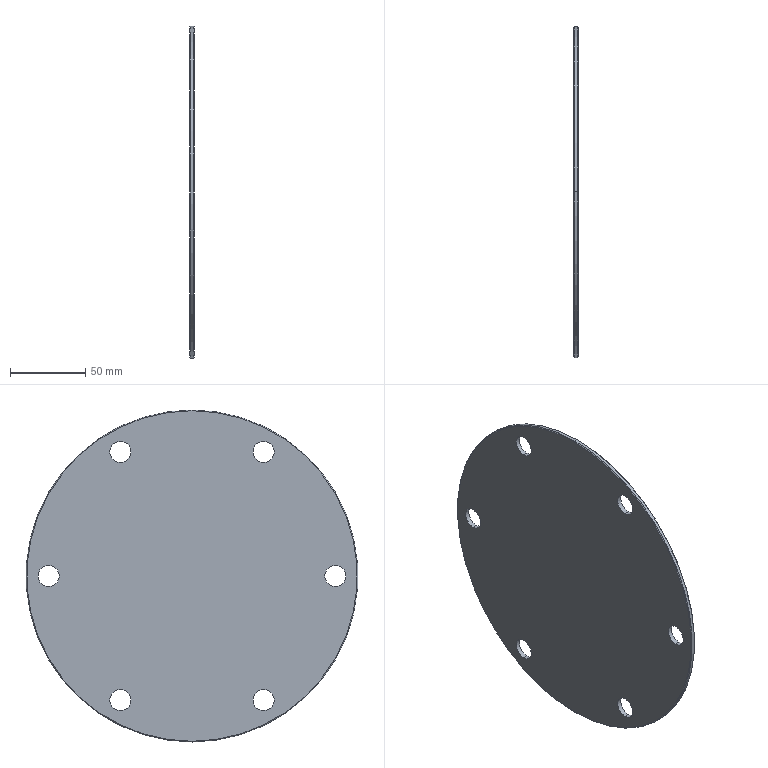Component | SolidWorks | YC1-200-01-11BodySideCover-1 | 1 solid | 20 faces | box 3 x 220 x 220 mm | volume 111096 mm3 | cylinder 14 | cone 4 | plane 2 | commonest cylinder face diameters 14 x12 220 x2 | material Plain Carbon Steel
STEP:
#1=COLOUR_RGB('',0.7922,0.8196,0.9333);
#2=FILL_AREA_STYLE_COLOUR('',#1);
#3=FILL_AREA_STYLE('',(#2));
#4=SURFACE_STYLE_FILL_AREA(#3);
#5=SURFACE_SIDE_STYLE('',(#4));
#6=SURFACE_STYLE_USAGE(.BOTH.,#5);
#7=PRESENTATION_STYLE_ASSIGNMENT((#6));
#8=CARTESIAN_POINT('',(-26.378,131.693,-29.508));
#9=VERTEX_POINT('',#8);
#10=CARTESIAN_POINT('',(-26.378,131.693,-38.13));
#11=VERTEX_POINT('',#10);
#12=CARTESIAN_POINT('',(-26.378,131.693,-33.819));
#13=DIRECTION('',(-1.,0.,0.));
#14=DIRECTION('',(0.,0.,1.));
#15=AXIS2_PLACEMENT_3D('',#12,#13,#14);
#16=CIRCLE('',#15,4.311);
#17=EDGE_CURVE('',#9,#11,#16,.T.);
#18=ORIENTED_EDGE('',*,*,#17,.T.);
#19=CARTESIAN_POINT('',(-26.398,131.693,-38.15));
#20=VERTEX_POINT('',#19);
#21=CARTESIAN_POINT('',(-26.398,131.693,-38.15));
#22=DIRECTION('',(-0.7071,0.,-0.7071));
#23=VECTOR('',#22,39.37);
#24=LINE('',#21,#23);
#25=EDGE_CURVE('',#11,#20,#24,.T.);
#26=ORIENTED_EDGE('',*,*,#25,.T.);
#27=CARTESIAN_POINT('',(-26.398,131.693,-29.488));
#28=VERTEX_POINT('',#27);
#29=CARTESIAN_POINT('',(-26.398,131.693,-33.819));
#30=DIRECTION('',(1.,0.,0.));
#31=DIRECTION('',(0.,0.,1.));
#32=AXIS2_PLACEMENT_3D('',#29,#30,#31);
#33=CIRCLE('',#32,4.331);
#34=EDGE_CURVE('',#20,#28,#33,.T.);
#35=ORIENTED_EDGE('',*,*,#34,.T.);
#36=CARTESIAN_POINT('',(-26.398,131.693,-29.488));
#37=DIRECTION('',(-0.7071,0.,0.7071));
#38=VECTOR('',#37,39.37);
#39=LINE('',#36,#38);
#40=EDGE_CURVE('',#9,#28,#39,.T.);
#41=ORIENTED_EDGE('',*,*,#40,.F.);
#42=EDGE_LOOP('',(#18,#26,#35,#41));
#43=FACE_OUTER_BOUND('',#42,.T.);
#44=CARTESIAN_POINT('',(-26.398,131.693,-33.819));
#45=DIRECTION('',(-1.,0.,0.));
#46=DIRECTION('',(0.,0.,1.));
#47=AXIS2_PLACEMENT_3D('',#44,#45,#46);
#48=CONICAL_SURFACE('',#47,4.331,0.7854);
#49=ADVANCED_FACE('',(#43),#48,.T.);
#50=CARTESIAN_POINT('',(-26.378,133.563,-36.782));
#51=VERTEX_POINT('',#50);
#52=CARTESIAN_POINT('',(-26.378,133.563,-37.334));
#53=VERTEX_POINT('',#52);
#54=CARTESIAN_POINT('',(-26.378,133.563,-37.058));
#55=DIRECTION('',(1.,0.,0.));
#56=DIRECTION('',(0.,0.,1.));
#57=AXIS2_PLACEMENT_3D('',#54,#55,#56);
#58=CIRCLE('',#57,0.2756);
#59=EDGE_CURVE('',#51,#53,#58,.T.);
#60=ORIENTED_EDGE('',*,*,#59,.T.);
#61=CARTESIAN_POINT('',(-26.496,133.563,-37.334));
#62=VERTEX_POINT('',#61);
#63=CARTESIAN_POINT('',(-26.496,133.563,-37.334));
#64=DIRECTION('',(-1.,0.,0.));
#65=VECTOR('',#64,39.37);
#66=LINE('',#63,#65);
#67=EDGE_CURVE('',#53,#62,#66,.T.);
#68=ORIENTED_EDGE('',*,*,#67,.T.);
#69=CARTESIAN_POINT('',(-26.496,133.563,-36.782));
#70=VERTEX_POINT('',#69);
#71=CARTESIAN_POINT('',(-26.496,133.563,-37.058));
#72=DIRECTION('',(1.,0.,0.));
#73=DIRECTION('',(0.,0.,1.));
#74=AXIS2_PLACEMENT_3D('',#71,#72,#73);
#75=CIRCLE('',#74,0.2756);
#76=EDGE_CURVE('',#70,#62,#75,.T.);
#77=ORIENTED_EDGE('',*,*,#76,.F.);
#78=CARTESIAN_POINT('',(-26.496,133.563,-36.782));
#79=DIRECTION('',(-1.,0.,0.));
#80=VECTOR('',#79,39.37);
#81=LINE('',#78,#80);
#82=EDGE_CURVE('',#51,#70,#81,.T.);
#83=ORIENTED_EDGE('',*,*,#82,.F.);
#84=EDGE_LOOP('',(#60,#68,#77,#83));
#85=FACE_OUTER_BOUND('',#84,.T.);
#86=CARTESIAN_POINT('',(-26.496,133.563,-37.058));
#87=DIRECTION('',(-1.,0.,0.));
#88=DIRECTION('',(0.,0.,1.));
#89=AXIS2_PLACEMENT_3D('',#86,#87,#88);
#90=CYLINDRICAL_SURFACE('',#89,0.2756);
#91=ADVANCED_FACE('',(#85),#90,.F.);
#92=CARTESIAN_POINT('',(-26.378,129.823,-36.782));
#93=VERTEX_POINT('',#92);
#94=CARTESIAN_POINT('',(-26.378,129.823,-37.334));
#95=VERTEX_POINT('',#94);
#96=CARTESIAN_POINT('',(-26.378,129.823,-37.058));
#97=DIRECTION('',(1.,0.,0.));
#98=DIRECTION('',(0.,0.,1.));
#99=AXIS2_PLACEMENT_3D('',#96,#97,#98);
#100=CIRCLE('',#99,0.2756);
#101=EDGE_CURVE('',#93,#95,#100,.T.);
#102=ORIENTED_EDGE('',*,*,#101,.T.);
#103=CARTESIAN_POINT('',(-26.496,129.823,-37.334));
#104=VERTEX_POINT('',#103);
#105=CARTESIAN_POINT('',(-26.496,129.823,-37.334));
#106=DIRECTION('',(-1.,0.,0.));
#107=VECTOR('',#106,39.37);
#108=LINE('',#105,#107);
#109=EDGE_CURVE('',#95,#104,#108,.T.);
#110=ORIENTED_EDGE('',*,*,#109,.T.);
#111=CARTESIAN_POINT('',(-26.496,129.823,-36.782));
#112=VERTEX_POINT('',#111);
#113=CARTESIAN_POINT('',(-26.496,129.823,-37.058));
#114=DIRECTION('',(1.,0.,0.));
#115=DIRECTION('',(0.,0.,1.));
#116=AXIS2_PLACEMENT_3D('',#113,#114,#115);
#117=CIRCLE('',#116,0.2756);
#118=EDGE_CURVE('',#112,#104,#117,.T.);
#119=ORIENTED_EDGE('',*,*,#118,.F.);
#120=CARTESIAN_POINT('',(-26.496,129.823,-36.782));
#121=DIRECTION('',(-1.,0.,0.));
#122=VECTOR('',#121,39.37);
#123=LINE('',#120,#122);
#124=EDGE_CURVE('',#93,#112,#123,.T.);
#125=ORIENTED_EDGE('',*,*,#124,.F.);
#126=EDGE_LOOP('',(#102,#110,#119,#125));
#127=FACE_OUTER_BOUND('',#126,.T.);
#128=CARTESIAN_POINT('',(-26.496,129.823,-37.058));
#129=DIRECTION('',(-1.,0.,0.));
#130=DIRECTION('',(0.,0.,1.));
#131=AXIS2_PLACEMENT_3D('',#128,#129,#130);
#132=CYLINDRICAL_SURFACE('',#131,0.2756);
#133=ADVANCED_FACE('',(#127),#132,.F.);
#134=CARTESIAN_POINT('',(-26.378,127.953,-33.543));
#135=VERTEX_POINT('',#134);
#136=CARTESIAN_POINT('',(-26.378,127.953,-34.094));
#137=VERTEX_POINT('',#136);
#138=CARTESIAN_POINT('',(-26.378,127.953,-33.819));
#139=DIRECTION('',(1.,0.,0.));
#140=DIRECTION('',(0.,0.,1.));
#141=AXIS2_PLACEMENT_3D('',#138,#139,#140);
#142=CIRCLE('',#141,0.2756);
#143=EDGE_CURVE('',#135,#137,#142,.T.);
#144=ORIENTED_EDGE('',*,*,#143,.T.);
#145=CARTESIAN_POINT('',(-26.496,127.953,-34.094));
#146=VERTEX_POINT('',#145);
#147=CARTESIAN_POINT('',(-26.496,127.953,-34.094));
#148=DIRECTION('',(-1.,0.,0.));
#149=VECTOR('',#148,39.37);
#150=LINE('',#147,#149);
#151=EDGE_CURVE('',#137,#146,#150,.T.);
#152=ORIENTED_EDGE('',*,*,#151,.T.);
#153=CARTESIAN_POINT('',(-26.496,127.953,-33.543));
#154=VERTEX_POINT('',#153);
#155=CARTESIAN_POINT('',(-26.496,127.953,-33.819));
#156=DIRECTION('',(1.,0.,0.));
#157=DIRECTION('',(0.,0.,1.));
#158=AXIS2_PLACEMENT_3D('',#155,#156,#157);
#159=CIRCLE('',#158,0.2756);
#160=EDGE_CURVE('',#154,#146,#159,.T.);
#161=ORIENTED_EDGE('',*,*,#160,.F.);
#162=CARTESIAN_POINT('',(-26.496,127.953,-33.543));
#163=DIRECTION('',(-1.,0.,0.));
#164=VECTOR('',#163,39.37);
#165=LINE('',#162,#164);
#166=EDGE_CURVE('',#135,#154,#165,.T.);
#167=ORIENTED_EDGE('',*,*,#166,.F.);
#168=EDGE_LOOP('',(#144,#152,#161,#167));
#169=FACE_OUTER_BOUND('',#168,.T.);
#170=CARTESIAN_POINT('',(-26.496,127.953,-33.819));
#171=DIRECTION('',(-1.,0.,0.));
#172=DIRECTION('',(0.,0.,1.));
#173=AXIS2_PLACEMENT_3D('',#170,#171,#172);
#174=CYLINDRICAL_SURFACE('',#173,0.2756);
#175=ADVANCED_FACE('',(#169),#174,.F.);
#176=CARTESIAN_POINT('',(-26.378,129.823,-30.304));
#177=VERTEX_POINT('',#176);
#178=CARTESIAN_POINT('',(-26.378,129.823,-30.855));
#179=VERTEX_POINT('',#178);
#180=CARTESIAN_POINT('',(-26.378,129.823,-30.58));
#181=DIRECTION('',(1.,0.,0.));
#182=DIRECTION('',(0.,0.,1.));
#183=AXIS2_PLACEMENT_3D('',#180,#181,#182);
#184=CIRCLE('',#183,0.2756);
#185=EDGE_CURVE('',#177,#179,#184,.T.);
#186=ORIENTED_EDGE('',*,*,#185,.T.);
#187=CARTESIAN_POINT('',(-26.496,129.823,-30.855));
#188=VERTEX_POINT('',#187);
#189=CARTESIAN_POINT('',(-26.496,129.823,-30.855));
#190=DIRECTION('',(-1.,0.,0.));
#191=VECTOR('',#190,39.37);
#192=LINE('',#189,#191);
#193=EDGE_CURVE('',#179,#188,#192,.T.);
#194=ORIENTED_EDGE('',*,*,#193,.T.);
#195=CARTESIAN_POINT('',(-26.496,129.823,-30.304));
#196=VERTEX_POINT('',#195);
#197=CARTESIAN_POINT('',(-26.496,129.823,-30.58));
#198=DIRECTION('',(1.,0.,0.));
#199=DIRECTION('',(0.,0.,1.));
#200=AXIS2_PLACEMENT_3D('',#197,#198,#199);
#201=CIRCLE('',#200,0.2756);
#202=EDGE_CURVE('',#196,#188,#201,.T.);
#203=ORIENTED_EDGE('',*,*,#202,.F.);
#204=CARTESIAN_POINT('',(-26.496,129.823,-30.304));
#205=DIRECTION('',(-1.,0.,0.));
#206=VECTOR('',#205,39.37);
#207=LINE('',#204,#206);
#208=EDGE_CURVE('',#177,#196,#207,.T.);
#209=ORIENTED_EDGE('',*,*,#208,.F.);
#210=EDGE_LOOP('',(#186,#194,#203,#209));
#211=FACE_OUTER_BOUND('',#210,.T.);
#212=CARTESIAN_POINT('',(-26.496,129.823,-30.58));
#213=DIRECTION('',(-1.,0.,0.));
#214=DIRECTION('',(0.,0.,1.));
#215=AXIS2_PLACEMENT_3D('',#212,#213,#214);
#216=CYLINDRICAL_SURFACE('',#215,0.2756);
#217=ADVANCED_FACE('',(#211),#216,.F.);
#218=CARTESIAN_POINT('',(-26.378,133.563,-30.304));
#219=VERTEX_POINT('',#218);
#220=CARTESIAN_POINT('',(-26.378,133.563,-30.855));
#221=VERTEX_POINT('',#220);
#222=CARTESIAN_POINT('',(-26.378,133.563,-30.58));
#223=DIRECTION('',(1.,0.,0.));
#224=DIRECTION('',(0.,0.,1.));
#225=AXIS2_PLACEMENT_3D('',#222,#223,#224);
#226=CIRCLE('',#225,0.2756);
#227=EDGE_CURVE('',#219,#221,#226,.T.);
#228=ORIENTED_EDGE('',*,*,#227,.T.);
#229=CARTESIAN_POINT('',(-26.496,133.563,-30.855));
#230=VERTEX_POINT('',#229);
#231=CARTESIAN_POINT('',(-26.496,133.563,-30.855));
#232=DIRECTION('',(-1.,0.,0.));
#233=VECTOR('',#232,39.37);
#234=LINE('',#231,#233);
#235=EDGE_CURVE('',#221,#230,#234,.T.);
#236=ORIENTED_EDGE('',*,*,#235,.T.);
#237=CARTESIAN_POINT('',(-26.496,133.563,-30.304));
#238=VERTEX_POINT('',#237);
#239=CARTESIAN_POINT('',(-26.496,133.563,-30.58));
#240=DIRECTION('',(1.,0.,0.));
#241=DIRECTION('',(0.,0.,1.));
#242=AXIS2_PLACEMENT_3D('',#239,#240,#241);
#243=CIRCLE('',#242,0.2756);
#244=EDGE_CURVE('',#238,#230,#243,.T.);
#245=ORIENTED_EDGE('',*,*,#244,.F.);
#246=CARTESIAN_POINT('',(-26.496,133.563,-30.304));
#247=DIRECTION('',(-1.,0.,0.));
#248=VECTOR('',#247,39.37);
#249=LINE('',#246,#248);
#250=EDGE_CURVE('',#219,#238,#249,.T.);
#251=ORIENTED_EDGE('',*,*,#250,.F.);
#252=EDGE_LOOP('',(#228,#236,#245,#251));
#253=FACE_OUTER_BOUND('',#252,.T.);
#254=CARTESIAN_POINT('',(-26.496,133.563,-30.58));
#255=DIRECTION('',(-1.,0.,0.));
#256=DIRECTION('',(0.,0.,1.));
#257=AXIS2_PLACEMENT_3D('',#254,#255,#256);
#258=CYLINDRICAL_SURFACE('',#257,0.2756);
#259=ADVANCED_FACE('',(#253),#258,.F.);
#260=CARTESIAN_POINT('',(-26.378,135.433,-33.543));
#261=VERTEX_POINT('',#260);
#262=CARTESIAN_POINT('',(-26.378,135.433,-34.094));
#263=VERTEX_POINT('',#262);
#264=CARTESIAN_POINT('',(-26.378,135.433,-33.819));
#265=DIRECTION('',(1.,0.,0.));
#266=DIRECTION('',(0.,0.,1.));
#267=AXIS2_PLACEMENT_3D('',#264,#265,#266);
#268=CIRCLE('',#267,0.2756);
#269=EDGE_CURVE('',#261,#263,#268,.T.);
#270=ORIENTED_EDGE('',*,*,#269,.T.);
#271=CARTESIAN_POINT('',(-26.496,135.433,-34.094));
#272=VERTEX_POINT('',#271);
#273=CARTESIAN_POINT('',(-26.496,135.433,-34.094));
#274=DIRECTION('',(-1.,0.,0.));
#275=VECTOR('',#274,39.37);
#276=LINE('',#273,#275);
#277=EDGE_CURVE('',#263,#272,#276,.T.);
#278=ORIENTED_EDGE('',*,*,#277,.T.);
#279=CARTESIAN_POINT('',(-26.496,135.433,-33.543));
#280=VERTEX_POINT('',#279);
#281=CARTESIAN_POINT('',(-26.496,135.433,-33.819));
#282=DIRECTION('',(1.,0.,0.));
#283=DIRECTION('',(0.,0.,1.));
#284=AXIS2_PLACEMENT_3D('',#281,#282,#283);
#285=CIRCLE('',#284,0.2756);
#286=EDGE_CURVE('',#280,#272,#285,.T.);
#287=ORIENTED_EDGE('',*,*,#286,.F.);
#288=CARTESIAN_POINT('',(-26.496,135.433,-33.543));
#289=DIRECTION('',(-1.,0.,0.));
#290=VECTOR('',#289,39.37);
#291=LINE('',#288,#290);
#292=EDGE_CURVE('',#261,#280,#291,.T.);
#293=ORIENTED_EDGE('',*,*,#292,.F.);
#294=EDGE_LOOP('',(#270,#278,#287,#293));
#295=FACE_OUTER_BOUND('',#294,.T.);
#296=CARTESIAN_POINT('',(-26.496,135.433,-33.819));
#297=DIRECTION('',(-1.,0.,0.));
#298=DIRECTION('',(0.,0.,1.));
#299=AXIS2_PLACEMENT_3D('',#296,#297,#298);
#300=CYLINDRICAL_SURFACE('',#299,0.2756);
#301=ADVANCED_FACE('',(#295),#300,.F.);
#302=ORIENTED_EDGE('',*,*,#34,.F.);
#303=CARTESIAN_POINT('',(-26.476,131.693,-38.15));
#304=VERTEX_POINT('',#303);
#305=CARTESIAN_POINT('',(-26.496,131.693,-38.15));
#306=DIRECTION('',(-1.,0.,0.));
#307=VECTOR('',#306,39.37);
#308=LINE('',#305,#307);
#309=EDGE_CURVE('',#20,#304,#308,.T.);
#310=ORIENTED_EDGE('',*,*,#309,.T.);
#311=CARTESIAN_POINT('',(-26.476,131.693,-29.488));
#312=VERTEX_POINT('',#311);
#313=CARTESIAN_POINT('',(-26.476,131.693,-33.819));
#314=DIRECTION('',(1.,0.,0.));
#315=DIRECTION('',(0.,0.,1.));
#316=AXIS2_PLACEMENT_3D('',#313,#314,#315);
#317=CIRCLE('',#316,4.331);
#318=EDGE_CURVE('',#304,#312,#317,.T.);
#319=ORIENTED_EDGE('',*,*,#318,.T.);
#320=CARTESIAN_POINT('',(-26.496,131.693,-29.488));
#321=DIRECTION('',(-1.,0.,0.));
#322=VECTOR('',#321,39.37);
#323=LINE('',#320,#322);
#324=EDGE_CURVE('',#28,#312,#323,.T.);
#325=ORIENTED_EDGE('',*,*,#324,.F.);
#326=EDGE_LOOP('',(#302,#310,#319,#325));
#327=FACE_OUTER_BOUND('',#326,.T.);
#328=CARTESIAN_POINT('',(-26.496,131.693,-33.819));
#329=DIRECTION('',(-1.,0.,0.));
#330=DIRECTION('',(0.,0.,1.));
#331=AXIS2_PLACEMENT_3D('',#328,#329,#330);
#332=CYLINDRICAL_SURFACE('',#331,4.331);
#333=ADVANCED_FACE('',(#327),#332,.T.);
#334=CARTESIAN_POINT('',(-26.496,131.693,-38.13));
#335=VERTEX_POINT('',#334);
#336=CARTESIAN_POINT('',(-26.496,131.693,-29.508));
#337=VERTEX_POINT('',#336);
#338=CARTESIAN_POINT('',(-26.496,131.693,-33.819));
#339=DIRECTION('',(1.,0.,0.));
#340=DIRECTION('',(0.,0.,-1.));
#341=AXIS2_PLACEMENT_3D('',#338,#339,#340);
#342=CIRCLE('',#341,4.311);
#343=EDGE_CURVE('',#335,#337,#342,.T.);
#344=ORIENTED_EDGE('',*,*,#343,.T.);
#345=CARTESIAN_POINT('',(-26.476,131.693,-29.488));
#346=DIRECTION('',(0.7071,0.,0.7071));
#347=VECTOR('',#346,39.37);
#348=LINE('',#345,#347);
#349=EDGE_CURVE('',#337,#312,#348,.T.);
#350=ORIENTED_EDGE('',*,*,#349,.T.);
#351=ORIENTED_EDGE('',*,*,#318,.F.);
#352=CARTESIAN_POINT('',(-26.476,131.693,-38.15));
#353=DIRECTION('',(0.7071,0.,-0.7071));
#354=VECTOR('',#353,39.37);
#355=LINE('',#352,#354);
#356=EDGE_CURVE('',#335,#304,#355,.T.);
#357=ORIENTED_EDGE('',*,*,#356,.F.);
#358=EDGE_LOOP('',(#344,#350,#351,#357));
#359=FACE_OUTER_BOUND('',#358,.T.);
#360=CARTESIAN_POINT('',(-26.476,131.693,-33.819));
#361=DIRECTION('',(1.,0.,0.));
#362=DIRECTION('',(0.,0.,-1.));
#363=AXIS2_PLACEMENT_3D('',#360,#361,#362);
#364=CONICAL_SURFACE('',#363,4.331,0.7854);
#365=ADVANCED_FACE('',(#359),#364,.T.);
#366=ORIENTED_EDGE('',*,*,#17,.F.);
#367=CARTESIAN_POINT('',(-26.378,131.693,-33.819));
#368=DIRECTION('',(-1.,0.,0.));
#369=DIRECTION('',(0.,0.,1.));
#370=AXIS2_PLACEMENT_3D('',#367,#368,#369);
#371=CIRCLE('',#370,4.311);
#372=EDGE_CURVE('',#11,#9,#371,.T.);
#373=ORIENTED_EDGE('',*,*,#372,.F.);
#374=EDGE_LOOP('',(#366,#373));
#375=FACE_OUTER_BOUND('',#374,.T.);
#376=ORIENTED_EDGE('',*,*,#59,.F.);
#377=CARTESIAN_POINT('',(-26.378,133.563,-37.058));
#378=DIRECTION('',(1.,0.,0.));
#379=DIRECTION('',(0.,0.,1.));
#380=AXIS2_PLACEMENT_3D('',#377,#378,#379);
#381=CIRCLE('',#380,0.2756);
#382=EDGE_CURVE('',#53,#51,#381,.T.);
#383=ORIENTED_EDGE('',*,*,#382,.F.);
#384=EDGE_LOOP('',(#376,#383));
#385=FACE_BOUND('',#384,.T.);
#386=ORIENTED_EDGE('',*,*,#101,.F.);
#387=CARTESIAN_POINT('',(-26.378,129.823,-37.058));
#388=DIRECTION('',(1.,0.,0.));
#389=DIRECTION('',(0.,0.,1.));
#390=AXIS2_PLACEMENT_3D('',#387,#388,#389);
#391=CIRCLE('',#390,0.2756);
#392=EDGE_CURVE('',#95,#93,#391,.T.);
#393=ORIENTED_EDGE('',*,*,#392,.F.);
#394=EDGE_LOOP('',(#386,#393));
#395=FACE_BOUND('',#394,.T.);
#396=ORIENTED_EDGE('',*,*,#143,.F.);
#397=CARTESIAN_POINT('',(-26.378,127.953,-33.819));
#398=DIRECTION('',(1.,0.,0.));
#399=DIRECTION('',(0.,0.,1.));
#400=AXIS2_PLACEMENT_3D('',#397,#398,#399);
#401=CIRCLE('',#400,0.2756);
#402=EDGE_CURVE('',#137,#135,#401,.T.);
#403=ORIENTED_EDGE('',*,*,#402,.F.);
#404=EDGE_LOOP('',(#396,#403));
#405=FACE_BOUND('',#404,.T.);
#406=ORIENTED_EDGE('',*,*,#185,.F.);
#407=CARTESIAN_POINT('',(-26.378,129.823,-30.58));
#408=DIRECTION('',(1.,0.,0.));
#409=DIRECTION('',(0.,0.,1.));
#410=AXIS2_PLACEMENT_3D('',#407,#408,#409);
#411=CIRCLE('',#410,0.2756);
#412=EDGE_CURVE('',#179,#177,#411,.T.);
#413=ORIENTED_EDGE('',*,*,#412,.F.);
#414=EDGE_LOOP('',(#406,#413));
#415=FACE_BOUND('',#414,.T.);
#416=ORIENTED_EDGE('',*,*,#227,.F.);
#417=CARTESIAN_POINT('',(-26.378,133.563,-30.58));
#418=DIRECTION('',(1.,0.,0.));
#419=DIRECTION('',(0.,0.,1.));
#420=AXIS2_PLACEMENT_3D('',#417,#418,#419);
#421=CIRCLE('',#420,0.2756);
#422=EDGE_CURVE('',#221,#219,#421,.T.);
#423=ORIENTED_EDGE('',*,*,#422,.F.);
#424=EDGE_LOOP('',(#416,#423));
#425=FACE_BOUND('',#424,.T.);
#426=ORIENTED_EDGE('',*,*,#269,.F.);
#427=CARTESIAN_POINT('',(-26.378,135.433,-33.819));
#428=DIRECTION('',(1.,0.,0.));
#429=DIRECTION('',(0.,0.,1.));
#430=AXIS2_PLACEMENT_3D('',#427,#428,#429);
#431=CIRCLE('',#430,0.2756);
#432=EDGE_CURVE('',#263,#261,#431,.T.);
#433=ORIENTED_EDGE('',*,*,#432,.F.);
#434=EDGE_LOOP('',(#426,#433));
#435=FACE_BOUND('',#434,.T.);
#436=CARTESIAN_POINT('',(-26.378,136.024,-33.819));
#437=DIRECTION('',(-1.,0.,0.));
#438=DIRECTION('',(0.,0.,1.));
#439=AXIS2_PLACEMENT_3D('',#436,#437,#438);
#440=PLANE('',#439);
#441=ADVANCED_FACE('',(#375,#385,#395,#405,#415,#425,#435),#440,.F.);
#442=ORIENTED_EDGE('',*,*,#25,.F.);
#443=ORIENTED_EDGE('',*,*,#372,.T.);
#444=ORIENTED_EDGE('',*,*,#40,.T.);
#445=CARTESIAN_POINT('',(-26.398,131.693,-33.819));
#446=DIRECTION('',(1.,0.,0.));
#447=DIRECTION('',(0.,0.,1.));
#448=AXIS2_PLACEMENT_3D('',#445,#446,#447);
#449=CIRCLE('',#448,4.331);
#450=EDGE_CURVE('',#28,#20,#449,.T.);
#451=ORIENTED_EDGE('',*,*,#450,.T.);
#452=EDGE_LOOP('',(#442,#443,#444,#451));
#453=FACE_OUTER_BOUND('',#452,.T.);
#454=CARTESIAN_POINT('',(-26.398,131.693,-33.819));
#455=DIRECTION('',(-1.,0.,0.));
#456=DIRECTION('',(0.,0.,1.));
#457=AXIS2_PLACEMENT_3D('',#454,#455,#456);
#458=CONICAL_SURFACE('',#457,4.331,0.7854);
#459=ADVANCED_FACE('',(#453),#458,.T.);
#460=ORIENTED_EDGE('',*,*,#67,.F.);
#461=ORIENTED_EDGE('',*,*,#382,.T.);
#462=ORIENTED_EDGE('',*,*,#82,.T.);
#463=CARTESIAN_POINT('',(-26.496,133.563,-37.058));
#464=DIRECTION('',(1.,0.,0.));
#465=DIRECTION('',(0.,0.,1.));
#466=AXIS2_PLACEMENT_3D('',#463,#464,#465);
#467=CIRCLE('',#466,0.2756);
#468=EDGE_CURVE('',#62,#70,#467,.T.);
#469=ORIENTED_EDGE('',*,*,#468,.F.);
#470=EDGE_LOOP('',(#460,#461,#462,#469));
#471=FACE_OUTER_BOUND('',#470,.T.);
#472=CARTESIAN_POINT('',(-26.496,133.563,-37.058));
#473=DIRECTION('',(-1.,0.,0.));
#474=DIRECTION('',(0.,0.,1.));
#475=AXIS2_PLACEMENT_3D('',#472,#473,#474);
#476=CYLINDRICAL_SURFACE('',#475,0.2756);
#477=ADVANCED_FACE('',(#471),#476,.F.);
#478=ORIENTED_EDGE('',*,*,#109,.F.);
#479=ORIENTED_EDGE('',*,*,#392,.T.);
#480=ORIENTED_EDGE('',*,*,#124,.T.);
#481=CARTESIAN_POINT('',(-26.496,129.823,-37.058));
#482=DIRECTION('',(1.,0.,0.));
#483=DIRECTION('',(0.,0.,1.));
#484=AXIS2_PLACEMENT_3D('',#481,#482,#483);
#485=CIRCLE('',#484,0.2756);
#486=EDGE_CURVE('',#104,#112,#485,.T.);
#487=ORIENTED_EDGE('',*,*,#486,.F.);
#488=EDGE_LOOP('',(#478,#479,#480,#487));
#489=FACE_OUTER_BOUND('',#488,.T.);
#490=CARTESIAN_POINT('',(-26.496,129.823,-37.058));
#491=DIRECTION('',(-1.,0.,0.));
#492=DIRECTION('',(0.,0.,1.));
#493=AXIS2_PLACEMENT_3D('',#490,#491,#492);
#494=CYLINDRICAL_SURFACE('',#493,0.2756);
#495=ADVANCED_FACE('',(#489),#494,.F.);
#496=ORIENTED_EDGE('',*,*,#151,.F.);
#497=ORIENTED_EDGE('',*,*,#402,.T.);
#498=ORIENTED_EDGE('',*,*,#166,.T.);
#499=CARTESIAN_POINT('',(-26.496,127.953,-33.819));
#500=DIRECTION('',(1.,0.,0.));
#501=DIRECTION('',(0.,0.,1.));
#502=AXIS2_PLACEMENT_3D('',#499,#500,#501);
#503=CIRCLE('',#502,0.2756);
#504=EDGE_CURVE('',#146,#154,#503,.T.);
#505=ORIENTED_EDGE('',*,*,#504,.F.);
#506=EDGE_LOOP('',(#496,#497,#498,#505));
#507=FACE_OUTER_BOUND('',#506,.T.);
#508=CARTESIAN_POINT('',(-26.496,127.953,-33.819));
#509=DIRECTION('',(-1.,0.,0.));
#510=DIRECTION('',(0.,0.,1.));
#511=AXIS2_PLACEMENT_3D('',#508,#509,#510);
#512=CYLINDRICAL_SURFACE('',#511,0.2756);
#513=ADVANCED_FACE('',(#507),#512,.F.);
#514=ORIENTED_EDGE('',*,*,#193,.F.);
#515=ORIENTED_EDGE('',*,*,#412,.T.);
#516=ORIENTED_EDGE('',*,*,#208,.T.);
#517=CARTESIAN_POINT('',(-26.496,129.823,-30.58));
#518=DIRECTION('',(1.,0.,0.));
#519=DIRECTION('',(0.,0.,1.));
#520=AXIS2_PLACEMENT_3D('',#517,#518,#519);
#521=CIRCLE('',#520,0.2756);
#522=EDGE_CURVE('',#188,#196,#521,.T.);
#523=ORIENTED_EDGE('',*,*,#522,.F.);
#524=EDGE_LOOP('',(#514,#515,#516,#523));
#525=FACE_OUTER_BOUND('',#524,.T.);
#526=CARTESIAN_POINT('',(-26.496,129.823,-30.58));
#527=DIRECTION('',(-1.,0.,0.));
#528=DIRECTION('',(0.,0.,1.));
#529=AXIS2_PLACEMENT_3D('',#526,#527,#528);
#530=CYLINDRICAL_SURFACE('',#529,0.2756);
#531=ADVANCED_FACE('',(#525),#530,.F.);
#532=ORIENTED_EDGE('',*,*,#235,.F.);
#533=ORIENTED_EDGE('',*,*,#422,.T.);
#534=ORIENTED_EDGE('',*,*,#250,.T.);
#535=CARTESIAN_POINT('',(-26.496,133.563,-30.58));
#536=DIRECTION('',(1.,0.,0.));
#537=DIRECTION('',(0.,0.,1.));
#538=AXIS2_PLACEMENT_3D('',#535,#536,#537);
#539=CIRCLE('',#538,0.2756);
#540=EDGE_CURVE('',#230,#238,#539,.T.);
#541=ORIENTED_EDGE('',*,*,#540,.F.);
#542=EDGE_LOOP('',(#532,#533,#534,#541));
#543=FACE_OUTER_BOUND('',#542,.T.);
#544=CARTESIAN_POINT('',(-26.496,133.563,-30.58));
#545=DIRECTION('',(-1.,0.,0.));
#546=DIRECTION('',(0.,0.,1.));
#547=AXIS2_PLACEMENT_3D('',#544,#545,#546);
#548=CYLINDRICAL_SURFACE('',#547,0.2756);
#549=ADVANCED_FACE('',(#543),#548,.F.);
#550=ORIENTED_EDGE('',*,*,#277,.F.);
#551=ORIENTED_EDGE('',*,*,#432,.T.);
#552=ORIENTED_EDGE('',*,*,#292,.T.);
#553=CARTESIAN_POINT('',(-26.496,135.433,-33.819));
#554=DIRECTION('',(1.,0.,0.));
#555=DIRECTION('',(0.,0.,1.));
#556=AXIS2_PLACEMENT_3D('',#553,#554,#555);
#557=CIRCLE('',#556,0.2756);
#558=EDGE_CURVE('',#272,#280,#557,.T.);
#559=ORIENTED_EDGE('',*,*,#558,.F.);
#560=EDGE_LOOP('',(#550,#551,#552,#559));
#561=FACE_OUTER_BOUND('',#560,.T.);
#562=CARTESIAN_POINT('',(-26.496,135.433,-33.819));
#563=DIRECTION('',(-1.,0.,0.));
#564=DIRECTION('',(0.,0.,1.));
#565=AXIS2_PLACEMENT_3D('',#562,#563,#564);
#566=CYLINDRICAL_SURFACE('',#565,0.2756);
#567=ADVANCED_FACE('',(#561),#566,.F.);
#568=ORIENTED_EDGE('',*,*,#309,.F.);
#569=ORIENTED_EDGE('',*,*,#450,.F.);
#570=ORIENTED_EDGE('',*,*,#324,.T.);
#571=CARTESIAN_POINT('',(-26.476,131.693,-33.819));
#572=DIRECTION('',(1.,0.,0.));
#573=DIRECTION('',(0.,0.,1.));
#574=AXIS2_PLACEMENT_3D('',#571,#572,#573);
#575=CIRCLE('',#574,4.331);
#576=EDGE_CURVE('',#312,#304,#575,.T.);
#577=ORIENTED_EDGE('',*,*,#576,.T.);
#578=EDGE_LOOP('',(#568,#569,#570,#577));
#579=FACE_OUTER_BOUND('',#578,.T.);
#580=CARTESIAN_POINT('',(-26.496,131.693,-33.819));
#581=DIRECTION('',(-1.,0.,0.));
#582=DIRECTION('',(0.,0.,1.));
#583=AXIS2_PLACEMENT_3D('',#580,#581,#582);
#584=CYLINDRICAL_SURFACE('',#583,4.331);
#585=ADVANCED_FACE('',(#579),#584,.T.);
#586=ORIENTED_EDGE('',*,*,#343,.F.);
#587=CARTESIAN_POINT('',(-26.496,131.693,-33.819));
#588=DIRECTION('',(1.,0.,0.));
#589=DIRECTION('',(0.,0.,-1.));
#590=AXIS2_PLACEMENT_3D('',#587,#588,#589);
#591=CIRCLE('',#590,4.311);
#592=EDGE_CURVE('',#337,#335,#591,.T.);
#593=ORIENTED_EDGE('',*,*,#592,.F.);
#594=EDGE_LOOP('',(#586,#593));
#595=FACE_OUTER_BOUND('',#594,.T.);
#596=ORIENTED_EDGE('',*,*,#76,.T.);
#597=ORIENTED_EDGE('',*,*,#468,.T.);
#598=EDGE_LOOP('',(#596,#597));
#599=FACE_BOUND('',#598,.T.);
#600=ORIENTED_EDGE('',*,*,#118,.T.);
#601=ORIENTED_EDGE('',*,*,#486,.T.);
#602=EDGE_LOOP('',(#600,#601));
#603=FACE_BOUND('',#602,.T.);
#604=ORIENTED_EDGE('',*,*,#160,.T.);
#605=ORIENTED_EDGE('',*,*,#504,.T.);
#606=EDGE_LOOP('',(#604,#605));
#607=FACE_BOUND('',#606,.T.);
#608=ORIENTED_EDGE('',*,*,#202,.T.);
#609=ORIENTED_EDGE('',*,*,#522,.T.);
#610=EDGE_LOOP('',(#608,#609));
#611=FACE_BOUND('',#610,.T.);
#612=ORIENTED_EDGE('',*,*,#244,.T.);
#613=ORIENTED_EDGE('',*,*,#540,.T.);
#614=EDGE_LOOP('',(#612,#613));
#615=FACE_BOUND('',#614,.T.);
#616=ORIENTED_EDGE('',*,*,#286,.T.);
#617=ORIENTED_EDGE('',*,*,#558,.T.);
#618=EDGE_LOOP('',(#616,#617));
#619=FACE_BOUND('',#618,.T.);
#620=CARTESIAN_POINT('',(-26.496,131.693,-33.819));
#621=DIRECTION('',(1.,0.,0.));
#622=DIRECTION('',(0.,0.,-1.));
#623=AXIS2_PLACEMENT_3D('',#620,#621,#622);
#624=PLANE('',#623);
#625=ADVANCED_FACE('',(#595,#599,#603,#607,#611,#615,#619),#624,.F.);
#626=ORIENTED_EDGE('',*,*,#349,.F.);
#627=ORIENTED_EDGE('',*,*,#592,.T.);
#628=ORIENTED_EDGE('',*,*,#356,.T.);
#629=ORIENTED_EDGE('',*,*,#576,.F.);
#630=EDGE_LOOP('',(#626,#627,#628,#629));
#631=FACE_OUTER_BOUND('',#630,.T.);
#632=CARTESIAN_POINT('',(-26.476,131.693,-33.819));
#633=DIRECTION('',(1.,0.,0.));
#634=DIRECTION('',(0.,0.,-1.));
#635=AXIS2_PLACEMENT_3D('',#632,#633,#634);
#636=CONICAL_SURFACE('',#635,4.331,0.7854);
#637=ADVANCED_FACE('',(#631),#636,.T.);
#638=CLOSED_SHELL('',(#49,#91,#133,#175,#217,#259,#301,#333,#365,#441,#459,#477,#495,#513,#531,#549,#567,#585,#625,#637));
#639=MANIFOLD_SOLID_BREP('',#638);
#640=STYLED_ITEM('',(#7),#639);
#641=PRESENTATION_LAYER_ASSIGNMENT('','',(#640));
#642=CARTESIAN_POINT('',(0.,0.,0.));
#643=DIRECTION('',(0.,0.,1.));
#644=DIRECTION('',(1.,0.,0.));
#645=AXIS2_PLACEMENT_3D('',#642,#643,#644);
#646=(LENGTH_UNIT()NAMED_UNIT(*)SI_UNIT($,.METRE.));
#647=LENGTH_MEASURE_WITH_UNIT(LENGTH_MEASURE(0.0254),#646);
#648=DIMENSIONAL_EXPONENTS(1.,0.,0.,0.,0.,0.,0.);
#649=(CONVERSION_BASED_UNIT('',#647)LENGTH_UNIT()NAMED_UNIT(#648));
#650=UNCERTAINTY_MEASURE_WITH_UNIT(LENGTH_MEASURE(0.00001),#649,'','');
#651=(NAMED_UNIT(*)PLANE_ANGLE_UNIT()SI_UNIT($,.RADIAN.));
#652=(NAMED_UNIT(*)SI_UNIT($,.STERADIAN.)SOLID_ANGLE_UNIT());
#653=(GEOMETRIC_REPRESENTATION_CONTEXT(3)GLOBAL_UNCERTAINTY_ASSIGNED_CONTEXT((#650))GLOBAL_UNIT_ASSIGNED_CONTEXT((#649,#651,#652))REPRESENTATION_CONTEXT('',''));
#654=ADVANCED_BREP_SHAPE_REPRESENTATION('',(#639,#645),#653);
#655=(LENGTH_UNIT()NAMED_UNIT(*)SI_UNIT($,.METRE.));
#656=LENGTH_MEASURE_WITH_UNIT(LENGTH_MEASURE(0.0254),#655);
#657=DIMENSIONAL_EXPONENTS(1.,0.,0.,0.,0.,0.,0.);
#658=(CONVERSION_BASED_UNIT('',#656)LENGTH_UNIT()NAMED_UNIT(#657));
#659=UNCERTAINTY_MEASURE_WITH_UNIT(LENGTH_MEASURE(0.00001),#658,'','');
#660=(NAMED_UNIT(*)PLANE_ANGLE_UNIT()SI_UNIT($,.RADIAN.));
#661=(NAMED_UNIT(*)SI_UNIT($,.STERADIAN.)SOLID_ANGLE_UNIT());
#662=(GEOMETRIC_REPRESENTATION_CONTEXT(3)GLOBAL_UNCERTAINTY_ASSIGNED_CONTEXT((#659))GLOBAL_UNIT_ASSIGNED_CONTEXT((#658,#660,#661))REPRESENTATION_CONTEXT('',''));
#663=MECHANICAL_DESIGN_GEOMETRIC_PRESENTATION_REPRESENTATION('',(#640),#662);